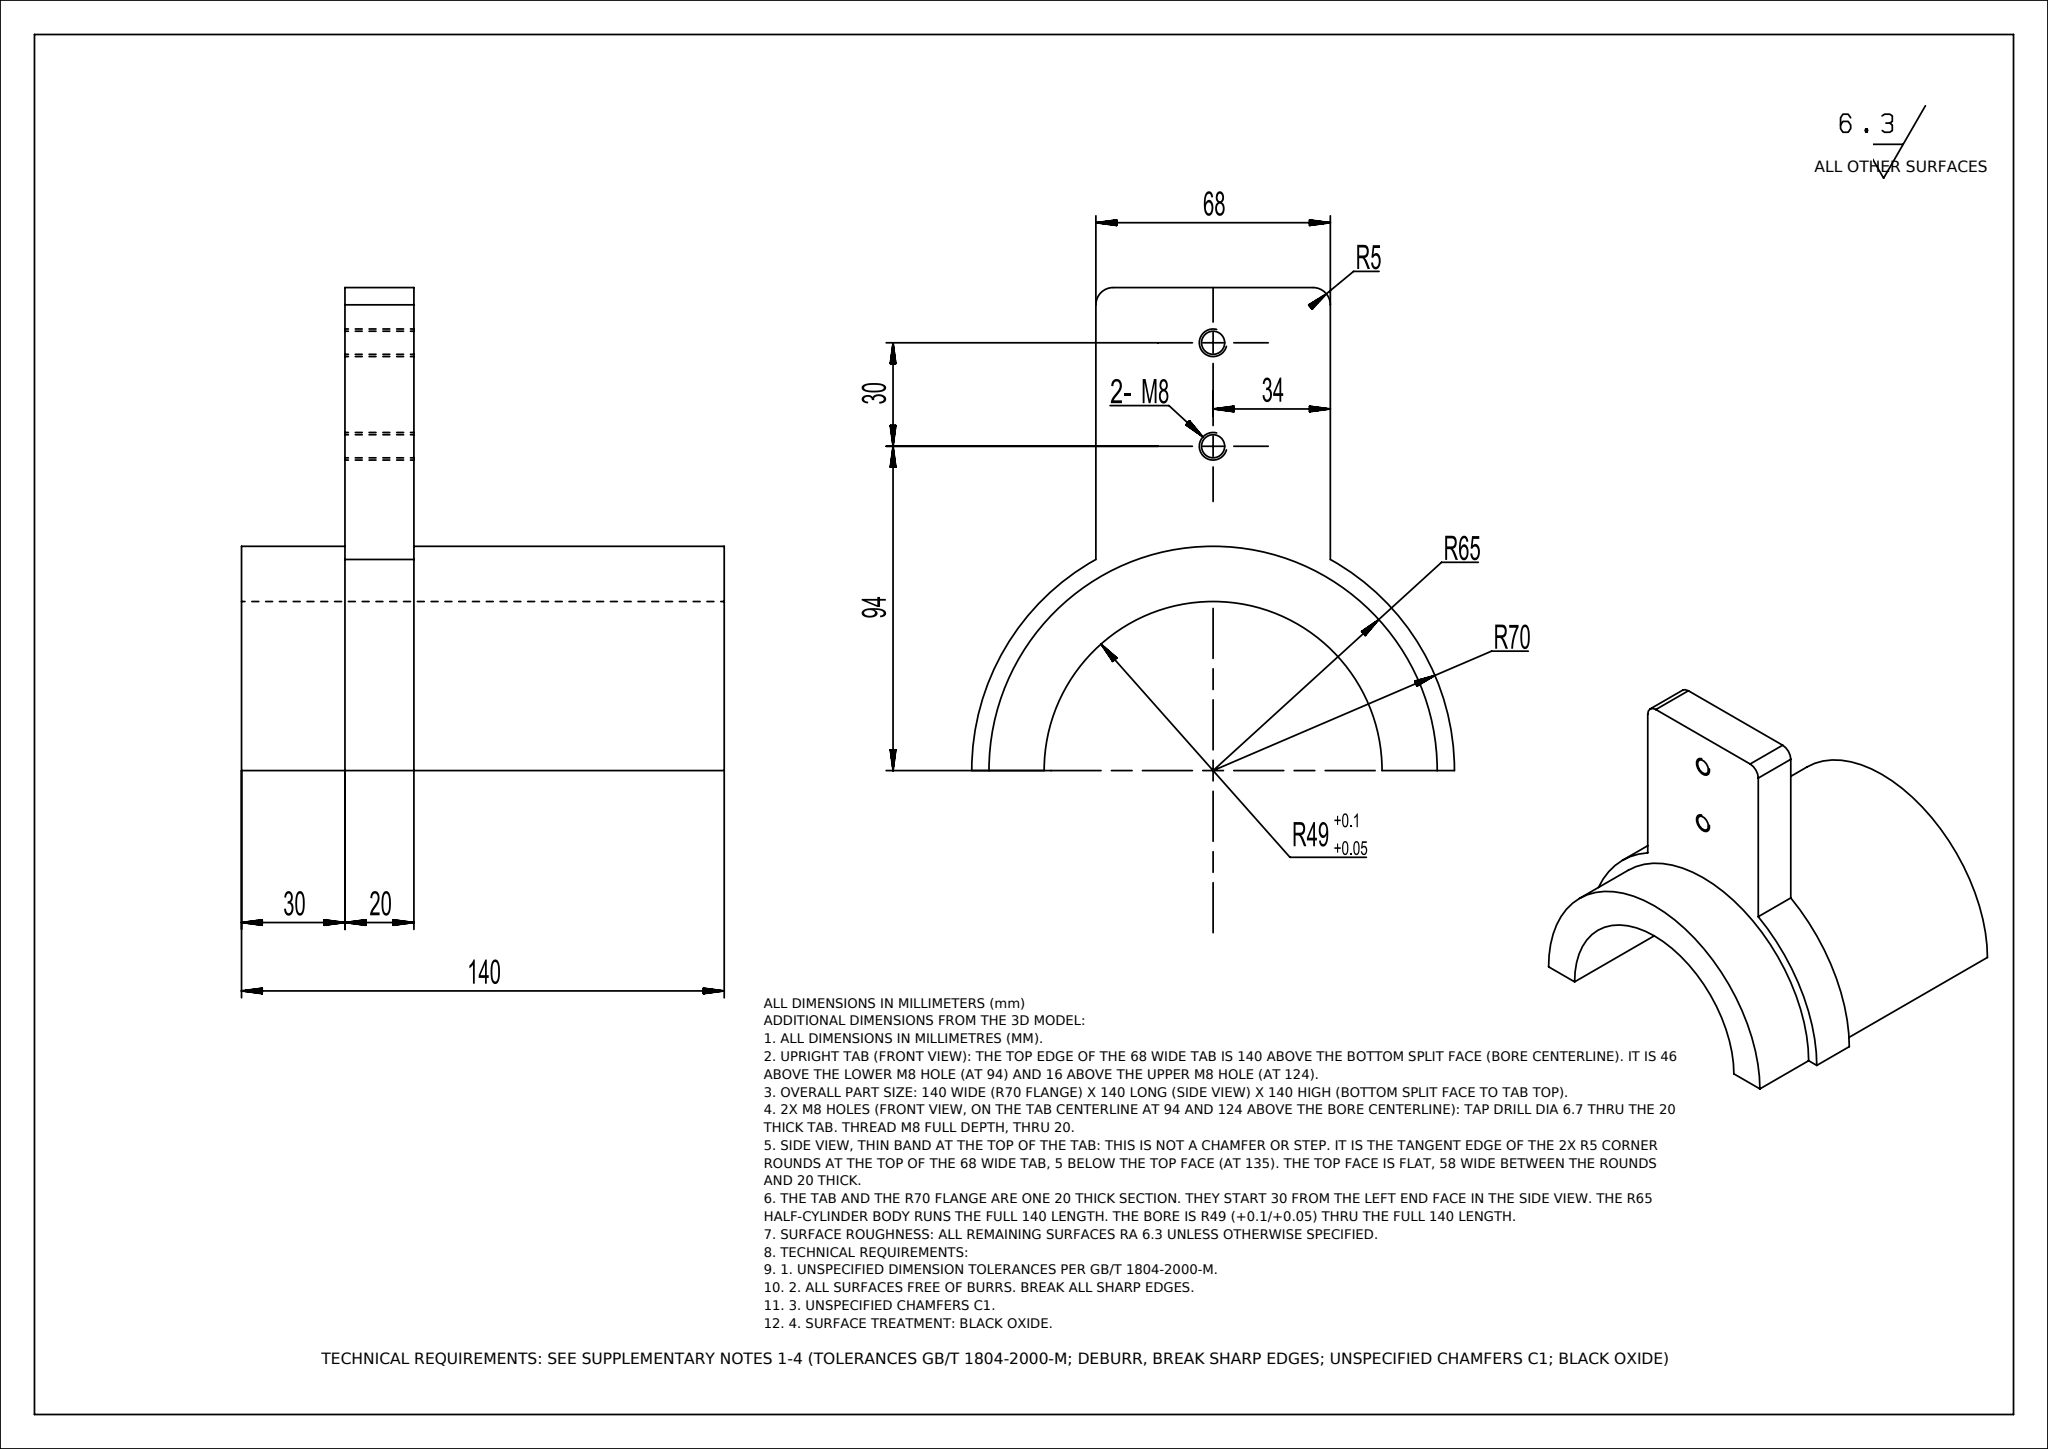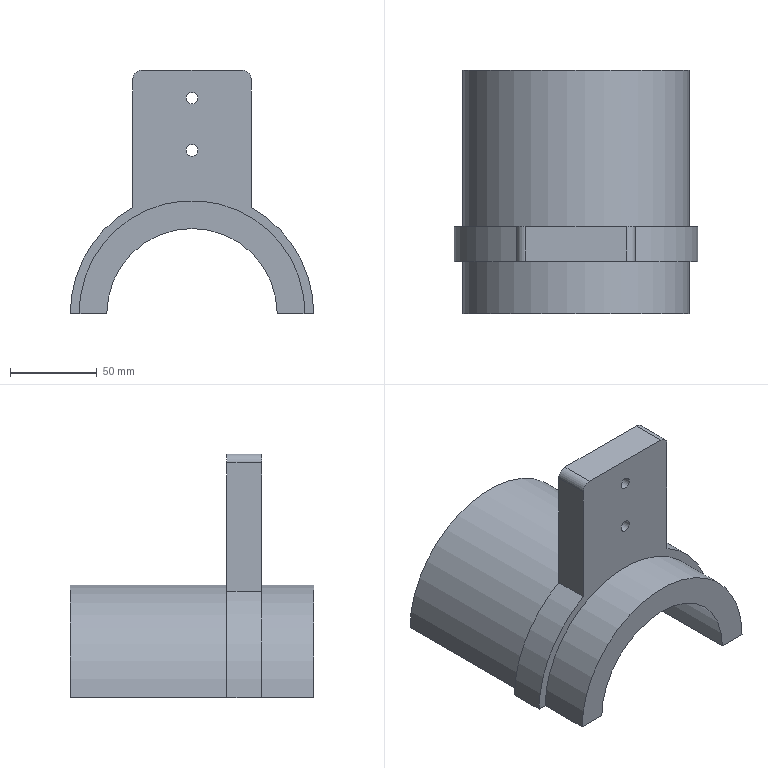Part | NX | mm | 1 solid | 18 faces | box 140 x 140 x 140 mm | volume 519788 mm3 | cylinder 9 | plane 9 | commonest cylinder face diameters 130 x2 140 x2 6.7 x2 10 x2 98 x1
STEP:
#1=CARTESIAN_POINT('',(0.,0.,0.));
#2=DIRECTION('',(0.,0.,1.));
#3=DIRECTION('',(1.,0.,0.));
#4=AXIS2_PLACEMENT_3D('',#1,#2,#3);
#5=(LENGTH_UNIT()NAMED_UNIT(*)SI_UNIT(.MILLI.,.METRE.));
#6=UNCERTAINTY_MEASURE_WITH_UNIT(LENGTH_MEASURE(0.00002),#5,'','');
#7=(NAMED_UNIT(*)PLANE_ANGLE_UNIT()SI_UNIT($,.RADIAN.));
#8=PLANE_ANGLE_MEASURE_WITH_UNIT(PLANE_ANGLE_MEASURE(0.01745),#7);
#9=DIMENSIONAL_EXPONENTS(0.,0.,0.,0.,0.,0.,0.);
#10=(CONVERSION_BASED_UNIT('',#8)NAMED_UNIT(#9)PLANE_ANGLE_UNIT());
#11=(NAMED_UNIT(*)SI_UNIT($,.STERADIAN.)SOLID_ANGLE_UNIT());
#12=(GEOMETRIC_REPRESENTATION_CONTEXT(3)GLOBAL_UNCERTAINTY_ASSIGNED_CONTEXT((#6))GLOBAL_UNIT_ASSIGNED_CONTEXT((#5,#10,#11))REPRESENTATION_CONTEXT('',''));
#13=SHAPE_REPRESENTATION('',(#4),#12);
#14=CARTESIAN_POINT('',(-65.,140.,0.));
#15=VERTEX_POINT('',#14);
#16=CARTESIAN_POINT('',(-65.,50.,0.));
#17=VERTEX_POINT('',#16);
#18=CARTESIAN_POINT('',(-65.,140.,0.));
#19=DIRECTION('',(0.,-1.,0.));
#20=VECTOR('',#19,1.);
#21=LINE('',#18,#20);
#22=EDGE_CURVE('',#15,#17,#21,.T.);
#23=ORIENTED_EDGE('',*,*,#22,.T.);
#24=CARTESIAN_POINT('',(65.,50.,0.));
#25=VERTEX_POINT('',#24);
#26=CARTESIAN_POINT('',(0.,50.,0.));
#27=DIRECTION('',(0.,1.,0.));
#28=DIRECTION('',(1.,0.,0.));
#29=AXIS2_PLACEMENT_3D('',#26,#27,#28);
#30=CIRCLE('',#29,65.);
#31=EDGE_CURVE('',#17,#25,#30,.T.);
#32=ORIENTED_EDGE('',*,*,#31,.T.);
#33=CARTESIAN_POINT('',(65.,140.,0.));
#34=VERTEX_POINT('',#33);
#35=CARTESIAN_POINT('',(65.,140.,0.));
#36=DIRECTION('',(0.,-1.,0.));
#37=VECTOR('',#36,1.);
#38=LINE('',#35,#37);
#39=EDGE_CURVE('',#34,#25,#38,.T.);
#40=ORIENTED_EDGE('',*,*,#39,.F.);
#41=CARTESIAN_POINT('',(0.,140.,0.));
#42=DIRECTION('',(0.,-1.,0.));
#43=DIRECTION('',(1.,0.,-0.));
#44=AXIS2_PLACEMENT_3D('',#41,#42,#43);
#45=CIRCLE('',#44,65.);
#46=EDGE_CURVE('',#34,#15,#45,.T.);
#47=ORIENTED_EDGE('',*,*,#46,.T.);
#48=EDGE_LOOP('',(#23,#32,#40,#47));
#49=FACE_OUTER_BOUND('',#48,.T.);
#50=CARTESIAN_POINT('',(0.,140.,0.));
#51=DIRECTION('',(0.,-1.,0.));
#52=DIRECTION('',(0.,0.,-1.));
#53=AXIS2_PLACEMENT_3D('',#50,#51,#52);
#54=CYLINDRICAL_SURFACE('',#53,65.);
#55=ADVANCED_FACE('',(#49),#54,.T.);
#56=CARTESIAN_POINT('',(-65.,0.,0.));
#57=VERTEX_POINT('',#56);
#58=CARTESIAN_POINT('',(-49.,0.,0.));
#59=VERTEX_POINT('',#58);
#60=CARTESIAN_POINT('',(-65.,0.,0.));
#61=DIRECTION('',(1.,0.,0.));
#62=VECTOR('',#61,1.);
#63=LINE('',#60,#62);
#64=EDGE_CURVE('',#57,#59,#63,.T.);
#65=ORIENTED_EDGE('',*,*,#64,.F.);
#66=CARTESIAN_POINT('',(-65.,30.,0.));
#67=VERTEX_POINT('',#66);
#68=CARTESIAN_POINT('',(-65.,140.,0.));
#69=DIRECTION('',(0.,-1.,0.));
#70=VECTOR('',#69,1.);
#71=LINE('',#68,#70);
#72=EDGE_CURVE('',#67,#57,#71,.T.);
#73=ORIENTED_EDGE('',*,*,#72,.F.);
#74=CARTESIAN_POINT('',(-70.,30.,0.));
#75=VERTEX_POINT('',#74);
#76=CARTESIAN_POINT('',(-70.,30.,0.));
#77=DIRECTION('',(1.,0.,0.));
#78=VECTOR('',#77,1.);
#79=LINE('',#76,#78);
#80=EDGE_CURVE('',#75,#67,#79,.T.);
#81=ORIENTED_EDGE('',*,*,#80,.F.);
#82=CARTESIAN_POINT('',(-70.,50.,0.));
#83=VERTEX_POINT('',#82);
#84=CARTESIAN_POINT('',(-70.,50.,0.));
#85=DIRECTION('',(0.,-1.,0.));
#86=VECTOR('',#85,1.);
#87=LINE('',#84,#86);
#88=EDGE_CURVE('',#83,#75,#87,.T.);
#89=ORIENTED_EDGE('',*,*,#88,.F.);
#90=CARTESIAN_POINT('',(-70.,50.,0.));
#91=DIRECTION('',(1.,0.,0.));
#92=VECTOR('',#91,1.);
#93=LINE('',#90,#92);
#94=EDGE_CURVE('',#83,#17,#93,.T.);
#95=ORIENTED_EDGE('',*,*,#94,.T.);
#96=ORIENTED_EDGE('',*,*,#22,.F.);
#97=CARTESIAN_POINT('',(-49.,140.,0.));
#98=VERTEX_POINT('',#97);
#99=CARTESIAN_POINT('',(-65.,140.,0.));
#100=DIRECTION('',(1.,0.,0.));
#101=VECTOR('',#100,1.);
#102=LINE('',#99,#101);
#103=EDGE_CURVE('',#15,#98,#102,.T.);
#104=ORIENTED_EDGE('',*,*,#103,.T.);
#105=CARTESIAN_POINT('',(-49.,140.,0.));
#106=DIRECTION('',(0.,-1.,0.));
#107=VECTOR('',#106,1.);
#108=LINE('',#105,#107);
#109=EDGE_CURVE('',#98,#59,#108,.T.);
#110=ORIENTED_EDGE('',*,*,#109,.T.);
#111=EDGE_LOOP('',(#65,#73,#81,#89,#95,#96,#104,#110));
#112=FACE_OUTER_BOUND('',#111,.T.);
#113=CARTESIAN_POINT('',(-65.,140.,0.));
#114=DIRECTION('',(0.,0.,-1.));
#115=DIRECTION('',(-1.,0.,-0.));
#116=AXIS2_PLACEMENT_3D('',#113,#114,#115);
#117=PLANE('',#116);
#118=ADVANCED_FACE('',(#112),#117,.T.);
#119=CARTESIAN_POINT('',(49.,0.,0.));
#120=VERTEX_POINT('',#119);
#121=CARTESIAN_POINT('',(0.,0.,0.));
#122=DIRECTION('',(0.,1.,0.));
#123=DIRECTION('',(1.,0.,0.));
#124=AXIS2_PLACEMENT_3D('',#121,#122,#123);
#125=CIRCLE('',#124,49.);
#126=EDGE_CURVE('',#59,#120,#125,.T.);
#127=ORIENTED_EDGE('',*,*,#126,.F.);
#128=ORIENTED_EDGE('',*,*,#109,.F.);
#129=CARTESIAN_POINT('',(49.,140.,0.));
#130=VERTEX_POINT('',#129);
#131=CARTESIAN_POINT('',(0.,140.,0.));
#132=DIRECTION('',(0.,1.,0.));
#133=DIRECTION('',(1.,0.,0.));
#134=AXIS2_PLACEMENT_3D('',#131,#132,#133);
#135=CIRCLE('',#134,49.);
#136=EDGE_CURVE('',#98,#130,#135,.T.);
#137=ORIENTED_EDGE('',*,*,#136,.T.);
#138=CARTESIAN_POINT('',(49.,140.,0.));
#139=DIRECTION('',(0.,-1.,0.));
#140=VECTOR('',#139,1.);
#141=LINE('',#138,#140);
#142=EDGE_CURVE('',#130,#120,#141,.T.);
#143=ORIENTED_EDGE('',*,*,#142,.T.);
#144=EDGE_LOOP('',(#127,#128,#137,#143));
#145=FACE_OUTER_BOUND('',#144,.T.);
#146=CARTESIAN_POINT('',(0.,140.,0.));
#147=DIRECTION('',(0.,-1.,0.));
#148=DIRECTION('',(0.,0.,-1.));
#149=AXIS2_PLACEMENT_3D('',#146,#147,#148);
#150=CYLINDRICAL_SURFACE('',#149,49.);
#151=ADVANCED_FACE('',(#145),#150,.F.);
#152=CARTESIAN_POINT('',(65.,0.,0.));
#153=VERTEX_POINT('',#152);
#154=CARTESIAN_POINT('',(49.,0.,0.));
#155=DIRECTION('',(1.,0.,0.));
#156=VECTOR('',#155,1.);
#157=LINE('',#154,#156);
#158=EDGE_CURVE('',#120,#153,#157,.T.);
#159=ORIENTED_EDGE('',*,*,#158,.F.);
#160=ORIENTED_EDGE('',*,*,#142,.F.);
#161=CARTESIAN_POINT('',(49.,140.,0.));
#162=DIRECTION('',(1.,0.,0.));
#163=VECTOR('',#162,1.);
#164=LINE('',#161,#163);
#165=EDGE_CURVE('',#130,#34,#164,.T.);
#166=ORIENTED_EDGE('',*,*,#165,.T.);
#167=ORIENTED_EDGE('',*,*,#39,.T.);
#168=CARTESIAN_POINT('',(70.,50.,-0.));
#169=VERTEX_POINT('',#168);
#170=CARTESIAN_POINT('',(65.,50.,0.));
#171=DIRECTION('',(1.,0.,-0.));
#172=VECTOR('',#171,1.);
#173=LINE('',#170,#172);
#174=EDGE_CURVE('',#25,#169,#173,.T.);
#175=ORIENTED_EDGE('',*,*,#174,.T.);
#176=CARTESIAN_POINT('',(70.,30.,-0.));
#177=VERTEX_POINT('',#176);
#178=CARTESIAN_POINT('',(70.,50.,-0.));
#179=DIRECTION('',(0.,-1.,0.));
#180=VECTOR('',#179,1.);
#181=LINE('',#178,#180);
#182=EDGE_CURVE('',#169,#177,#181,.T.);
#183=ORIENTED_EDGE('',*,*,#182,.T.);
#184=CARTESIAN_POINT('',(65.,30.,0.));
#185=VERTEX_POINT('',#184);
#186=CARTESIAN_POINT('',(65.,30.,0.));
#187=DIRECTION('',(1.,0.,-0.));
#188=VECTOR('',#187,1.);
#189=LINE('',#186,#188);
#190=EDGE_CURVE('',#185,#177,#189,.T.);
#191=ORIENTED_EDGE('',*,*,#190,.F.);
#192=CARTESIAN_POINT('',(65.,140.,0.));
#193=DIRECTION('',(0.,-1.,0.));
#194=VECTOR('',#193,1.);
#195=LINE('',#192,#194);
#196=EDGE_CURVE('',#185,#153,#195,.T.);
#197=ORIENTED_EDGE('',*,*,#196,.T.);
#198=EDGE_LOOP('',(#159,#160,#166,#167,#175,#183,#191,#197));
#199=FACE_OUTER_BOUND('',#198,.T.);
#200=CARTESIAN_POINT('',(49.,140.,0.));
#201=DIRECTION('',(0.,0.,-1.));
#202=DIRECTION('',(-1.,0.,-0.));
#203=AXIS2_PLACEMENT_3D('',#200,#201,#202);
#204=PLANE('',#203);
#205=ADVANCED_FACE('',(#199),#204,.T.);
#206=CARTESIAN_POINT('',(0.,30.,0.));
#207=DIRECTION('',(0.,1.,0.));
#208=DIRECTION('',(1.,0.,0.));
#209=AXIS2_PLACEMENT_3D('',#206,#207,#208);
#210=CIRCLE('',#209,65.);
#211=EDGE_CURVE('',#67,#185,#210,.T.);
#212=ORIENTED_EDGE('',*,*,#211,.F.);
#213=ORIENTED_EDGE('',*,*,#72,.T.);
#214=CARTESIAN_POINT('',(0.,0.,0.));
#215=DIRECTION('',(0.,-1.,0.));
#216=DIRECTION('',(1.,0.,-0.));
#217=AXIS2_PLACEMENT_3D('',#214,#215,#216);
#218=CIRCLE('',#217,65.);
#219=EDGE_CURVE('',#153,#57,#218,.T.);
#220=ORIENTED_EDGE('',*,*,#219,.F.);
#221=ORIENTED_EDGE('',*,*,#196,.F.);
#222=EDGE_LOOP('',(#212,#213,#220,#221));
#223=FACE_OUTER_BOUND('',#222,.T.);
#224=CARTESIAN_POINT('',(0.,140.,0.));
#225=DIRECTION('',(0.,-1.,0.));
#226=DIRECTION('',(0.,0.,-1.));
#227=AXIS2_PLACEMENT_3D('',#224,#225,#226);
#228=CYLINDRICAL_SURFACE('',#227,65.);
#229=ADVANCED_FACE('',(#223),#228,.T.);
#230=ORIENTED_EDGE('',*,*,#103,.F.);
#231=ORIENTED_EDGE('',*,*,#46,.F.);
#232=ORIENTED_EDGE('',*,*,#165,.F.);
#233=ORIENTED_EDGE('',*,*,#136,.F.);
#234=EDGE_LOOP('',(#230,#231,#232,#233));
#235=FACE_OUTER_BOUND('',#234,.T.);
#236=CARTESIAN_POINT('',(0.,140.,0.));
#237=DIRECTION('',(0.,1.,0.));
#238=DIRECTION('',(0.,0.,1.));
#239=AXIS2_PLACEMENT_3D('',#236,#237,#238);
#240=PLANE('',#239);
#241=ADVANCED_FACE('',(#235),#240,.T.);
#242=ORIENTED_EDGE('',*,*,#64,.T.);
#243=ORIENTED_EDGE('',*,*,#126,.T.);
#244=ORIENTED_EDGE('',*,*,#158,.T.);
#245=ORIENTED_EDGE('',*,*,#219,.T.);
#246=EDGE_LOOP('',(#242,#243,#244,#245));
#247=FACE_OUTER_BOUND('',#246,.T.);
#248=CARTESIAN_POINT('',(0.,0.,0.));
#249=DIRECTION('',(0.,1.,0.));
#250=DIRECTION('',(0.,0.,1.));
#251=AXIS2_PLACEMENT_3D('',#248,#249,#250);
#252=PLANE('',#251);
#253=ADVANCED_FACE('',(#247),#252,.F.);
#254=CARTESIAN_POINT('',(34.,30.,61.188));
#255=VERTEX_POINT('',#254);
#256=CARTESIAN_POINT('',(0.,30.,0.));
#257=DIRECTION('',(0.,-1.,0.));
#258=DIRECTION('',(1.,0.,-0.));
#259=AXIS2_PLACEMENT_3D('',#256,#257,#258);
#260=CIRCLE('',#259,70.);
#261=EDGE_CURVE('',#177,#255,#260,.T.);
#262=ORIENTED_EDGE('',*,*,#261,.F.);
#263=ORIENTED_EDGE('',*,*,#182,.F.);
#264=CARTESIAN_POINT('',(34.,50.,61.188));
#265=VERTEX_POINT('',#264);
#266=CARTESIAN_POINT('',(0.,50.,0.));
#267=DIRECTION('',(0.,-1.,0.));
#268=DIRECTION('',(1.,0.,-0.));
#269=AXIS2_PLACEMENT_3D('',#266,#267,#268);
#270=CIRCLE('',#269,70.);
#271=EDGE_CURVE('',#169,#265,#270,.T.);
#272=ORIENTED_EDGE('',*,*,#271,.T.);
#273=CARTESIAN_POINT('',(34.,50.,61.188));
#274=DIRECTION('',(0.,-1.,0.));
#275=VECTOR('',#274,1.);
#276=LINE('',#273,#275);
#277=EDGE_CURVE('',#265,#255,#276,.T.);
#278=ORIENTED_EDGE('',*,*,#277,.T.);
#279=EDGE_LOOP('',(#262,#263,#272,#278));
#280=FACE_OUTER_BOUND('',#279,.T.);
#281=CARTESIAN_POINT('',(0.,50.,0.));
#282=DIRECTION('',(0.,-1.,0.));
#283=DIRECTION('',(0.,0.,-1.));
#284=AXIS2_PLACEMENT_3D('',#281,#282,#283);
#285=CYLINDRICAL_SURFACE('',#284,70.);
#286=ADVANCED_FACE('',(#280),#285,.T.);
#287=CARTESIAN_POINT('',(34.,50.,135.));
#288=VERTEX_POINT('',#287);
#289=CARTESIAN_POINT('',(34.,50.,61.188));
#290=DIRECTION('',(-0.,0.,1.));
#291=VECTOR('',#290,1.);
#292=LINE('',#289,#291);
#293=EDGE_CURVE('',#265,#288,#292,.T.);
#294=ORIENTED_EDGE('',*,*,#293,.T.);
#295=CARTESIAN_POINT('',(34.,30.,135.));
#296=VERTEX_POINT('',#295);
#297=CARTESIAN_POINT('',(34.,50.,135.));
#298=DIRECTION('',(0.,-1.,0.));
#299=VECTOR('',#298,1.);
#300=LINE('',#297,#299);
#301=EDGE_CURVE('',#288,#296,#300,.T.);
#302=ORIENTED_EDGE('',*,*,#301,.T.);
#303=CARTESIAN_POINT('',(34.,30.,61.188));
#304=DIRECTION('',(-0.,0.,1.));
#305=VECTOR('',#304,1.);
#306=LINE('',#303,#305);
#307=EDGE_CURVE('',#255,#296,#306,.T.);
#308=ORIENTED_EDGE('',*,*,#307,.F.);
#309=ORIENTED_EDGE('',*,*,#277,.F.);
#310=EDGE_LOOP('',(#294,#302,#308,#309));
#311=FACE_OUTER_BOUND('',#310,.T.);
#312=CARTESIAN_POINT('',(34.,50.,61.188));
#313=DIRECTION('',(1.,0.,0.));
#314=DIRECTION('',(0.,0.,-1.));
#315=AXIS2_PLACEMENT_3D('',#312,#313,#314);
#316=PLANE('',#315);
#317=ADVANCED_FACE('',(#311),#316,.T.);
#318=CARTESIAN_POINT('',(29.,50.,140.));
#319=VERTEX_POINT('',#318);
#320=CARTESIAN_POINT('',(-29.,50.,140.));
#321=VERTEX_POINT('',#320);
#322=CARTESIAN_POINT('',(34.,50.,140.));
#323=DIRECTION('',(-1.,0.,0.));
#324=VECTOR('',#323,1.);
#325=LINE('',#322,#324);
#326=EDGE_CURVE('',#319,#321,#325,.T.);
#327=ORIENTED_EDGE('',*,*,#326,.T.);
#328=CARTESIAN_POINT('',(-29.,30.,140.));
#329=VERTEX_POINT('',#328);
#330=CARTESIAN_POINT('',(-29.,50.,140.));
#331=DIRECTION('',(0.,-1.,0.));
#332=VECTOR('',#331,1.);
#333=LINE('',#330,#332);
#334=EDGE_CURVE('',#321,#329,#333,.T.);
#335=ORIENTED_EDGE('',*,*,#334,.T.);
#336=CARTESIAN_POINT('',(29.,30.,140.));
#337=VERTEX_POINT('',#336);
#338=CARTESIAN_POINT('',(34.,30.,140.));
#339=DIRECTION('',(-1.,0.,0.));
#340=VECTOR('',#339,1.);
#341=LINE('',#338,#340);
#342=EDGE_CURVE('',#337,#329,#341,.T.);
#343=ORIENTED_EDGE('',*,*,#342,.F.);
#344=CARTESIAN_POINT('',(29.,50.,140.));
#345=DIRECTION('',(0.,1.,0.));
#346=VECTOR('',#345,1.);
#347=LINE('',#344,#346);
#348=EDGE_CURVE('',#337,#319,#347,.T.);
#349=ORIENTED_EDGE('',*,*,#348,.T.);
#350=EDGE_LOOP('',(#327,#335,#343,#349));
#351=FACE_OUTER_BOUND('',#350,.T.);
#352=CARTESIAN_POINT('',(34.,50.,140.));
#353=DIRECTION('',(0.,0.,1.));
#354=DIRECTION('',(1.,0.,0.));
#355=AXIS2_PLACEMENT_3D('',#352,#353,#354);
#356=PLANE('',#355);
#357=ADVANCED_FACE('',(#351),#356,.T.);
#358=CARTESIAN_POINT('',(-34.,30.,135.));
#359=VERTEX_POINT('',#358);
#360=CARTESIAN_POINT('',(-34.,30.,61.188));
#361=VERTEX_POINT('',#360);
#362=CARTESIAN_POINT('',(-34.,30.,140.));
#363=DIRECTION('',(-0.,0.,-1.));
#364=VECTOR('',#363,1.);
#365=LINE('',#362,#364);
#366=EDGE_CURVE('',#359,#361,#365,.T.);
#367=ORIENTED_EDGE('',*,*,#366,.F.);
#368=CARTESIAN_POINT('',(-34.,50.,135.));
#369=VERTEX_POINT('',#368);
#370=CARTESIAN_POINT('',(-34.,50.,135.));
#371=DIRECTION('',(0.,1.,0.));
#372=VECTOR('',#371,1.);
#373=LINE('',#370,#372);
#374=EDGE_CURVE('',#359,#369,#373,.T.);
#375=ORIENTED_EDGE('',*,*,#374,.T.);
#376=CARTESIAN_POINT('',(-34.,50.,61.188));
#377=VERTEX_POINT('',#376);
#378=CARTESIAN_POINT('',(-34.,50.,140.));
#379=DIRECTION('',(-0.,0.,-1.));
#380=VECTOR('',#379,1.);
#381=LINE('',#378,#380);
#382=EDGE_CURVE('',#369,#377,#381,.T.);
#383=ORIENTED_EDGE('',*,*,#382,.T.);
#384=CARTESIAN_POINT('',(-34.,50.,61.188));
#385=DIRECTION('',(0.,-1.,0.));
#386=VECTOR('',#385,1.);
#387=LINE('',#384,#386);
#388=EDGE_CURVE('',#377,#361,#387,.T.);
#389=ORIENTED_EDGE('',*,*,#388,.T.);
#390=EDGE_LOOP('',(#367,#375,#383,#389));
#391=FACE_OUTER_BOUND('',#390,.T.);
#392=CARTESIAN_POINT('',(-34.,50.,140.));
#393=DIRECTION('',(-1.,0.,0.));
#394=DIRECTION('',(0.,0.,1.));
#395=AXIS2_PLACEMENT_3D('',#392,#393,#394);
#396=PLANE('',#395);
#397=ADVANCED_FACE('',(#391),#396,.T.);
#398=CARTESIAN_POINT('',(3.35,50.,94.));
#399=VERTEX_POINT('',#398);
#400=CARTESIAN_POINT('',(0.,50.,94.));
#401=DIRECTION('',(0.,-1.,0.));
#402=DIRECTION('',(1.,0.,0.));
#403=AXIS2_PLACEMENT_3D('',#400,#401,#402);
#404=CIRCLE('',#403,3.35);
#405=EDGE_CURVE('',#399,#399,#404,.T.);
#406=ORIENTED_EDGE('',*,*,#405,.F.);
#407=EDGE_LOOP('',(#406));
#408=FACE_BOUND('',#407,.T.);
#409=CARTESIAN_POINT('',(3.35,30.,94.));
#410=VERTEX_POINT('',#409);
#411=CARTESIAN_POINT('',(0.,30.,94.));
#412=DIRECTION('',(0.,-1.,0.));
#413=DIRECTION('',(1.,0.,0.));
#414=AXIS2_PLACEMENT_3D('',#411,#412,#413);
#415=CIRCLE('',#414,3.35);
#416=EDGE_CURVE('',#410,#410,#415,.T.);
#417=ORIENTED_EDGE('',*,*,#416,.T.);
#418=EDGE_LOOP('',(#417));
#419=FACE_BOUND('',#418,.T.);
#420=CARTESIAN_POINT('',(0.,50.,94.));
#421=DIRECTION('',(0.,-1.,0.));
#422=DIRECTION('',(0.,0.,-1.));
#423=AXIS2_PLACEMENT_3D('',#420,#421,#422);
#424=CYLINDRICAL_SURFACE('',#423,3.35);
#425=ADVANCED_FACE('',(#408,#419),#424,.F.);
#426=CARTESIAN_POINT('',(0.,30.,0.));
#427=DIRECTION('',(0.,-1.,0.));
#428=DIRECTION('',(1.,0.,-0.));
#429=AXIS2_PLACEMENT_3D('',#426,#427,#428);
#430=CIRCLE('',#429,70.);
#431=EDGE_CURVE('',#361,#75,#430,.T.);
#432=ORIENTED_EDGE('',*,*,#431,.F.);
#433=ORIENTED_EDGE('',*,*,#388,.F.);
#434=CARTESIAN_POINT('',(0.,50.,0.));
#435=DIRECTION('',(0.,-1.,0.));
#436=DIRECTION('',(1.,0.,-0.));
#437=AXIS2_PLACEMENT_3D('',#434,#435,#436);
#438=CIRCLE('',#437,70.);
#439=EDGE_CURVE('',#377,#83,#438,.T.);
#440=ORIENTED_EDGE('',*,*,#439,.T.);
#441=ORIENTED_EDGE('',*,*,#88,.T.);
#442=EDGE_LOOP('',(#432,#433,#440,#441));
#443=FACE_OUTER_BOUND('',#442,.T.);
#444=CARTESIAN_POINT('',(0.,50.,0.));
#445=DIRECTION('',(0.,-1.,0.));
#446=DIRECTION('',(0.,0.,-1.));
#447=AXIS2_PLACEMENT_3D('',#444,#445,#446);
#448=CYLINDRICAL_SURFACE('',#447,70.);
#449=ADVANCED_FACE('',(#443),#448,.T.);
#450=CARTESIAN_POINT('',(3.35,50.,124.));
#451=VERTEX_POINT('',#450);
#452=CARTESIAN_POINT('',(0.,50.,124.));
#453=DIRECTION('',(0.,-1.,0.));
#454=DIRECTION('',(1.,0.,0.));
#455=AXIS2_PLACEMENT_3D('',#452,#453,#454);
#456=CIRCLE('',#455,3.35);
#457=EDGE_CURVE('',#451,#451,#456,.T.);
#458=ORIENTED_EDGE('',*,*,#457,.F.);
#459=EDGE_LOOP('',(#458));
#460=FACE_BOUND('',#459,.T.);
#461=CARTESIAN_POINT('',(3.35,30.,124.));
#462=VERTEX_POINT('',#461);
#463=CARTESIAN_POINT('',(0.,30.,124.));
#464=DIRECTION('',(0.,-1.,0.));
#465=DIRECTION('',(1.,0.,0.));
#466=AXIS2_PLACEMENT_3D('',#463,#464,#465);
#467=CIRCLE('',#466,3.35);
#468=EDGE_CURVE('',#462,#462,#467,.T.);
#469=ORIENTED_EDGE('',*,*,#468,.T.);
#470=EDGE_LOOP('',(#469));
#471=FACE_BOUND('',#470,.T.);
#472=CARTESIAN_POINT('',(0.,50.,124.));
#473=DIRECTION('',(0.,-1.,0.));
#474=DIRECTION('',(0.,0.,-1.));
#475=AXIS2_PLACEMENT_3D('',#472,#473,#474);
#476=CYLINDRICAL_SURFACE('',#475,3.35);
#477=ADVANCED_FACE('',(#460,#471),#476,.F.);
#478=ORIENTED_EDGE('',*,*,#382,.F.);
#479=CARTESIAN_POINT('',(-29.,50.,135.));
#480=DIRECTION('',(0.,1.,0.));
#481=DIRECTION('',(0.,0.,1.));
#482=AXIS2_PLACEMENT_3D('',#479,#480,#481);
#483=CIRCLE('',#482,5.);
#484=EDGE_CURVE('',#369,#321,#483,.T.);
#485=ORIENTED_EDGE('',*,*,#484,.T.);
#486=ORIENTED_EDGE('',*,*,#326,.F.);
#487=CARTESIAN_POINT('',(29.,50.,135.));
#488=DIRECTION('',(0.,1.,0.));
#489=DIRECTION('',(0.,0.,1.));
#490=AXIS2_PLACEMENT_3D('',#487,#488,#489);
#491=CIRCLE('',#490,5.);
#492=EDGE_CURVE('',#319,#288,#491,.T.);
#493=ORIENTED_EDGE('',*,*,#492,.T.);
#494=ORIENTED_EDGE('',*,*,#293,.F.);
#495=ORIENTED_EDGE('',*,*,#271,.F.);
#496=ORIENTED_EDGE('',*,*,#174,.F.);
#497=ORIENTED_EDGE('',*,*,#31,.F.);
#498=ORIENTED_EDGE('',*,*,#94,.F.);
#499=ORIENTED_EDGE('',*,*,#439,.F.);
#500=EDGE_LOOP('',(#478,#485,#486,#493,#494,#495,#496,#497,#498,#499));
#501=FACE_BOUND('',#500,.T.);
#502=ORIENTED_EDGE('',*,*,#405,.T.);
#503=EDGE_LOOP('',(#502));
#504=FACE_BOUND('',#503,.T.);
#505=ORIENTED_EDGE('',*,*,#457,.T.);
#506=EDGE_LOOP('',(#505));
#507=FACE_BOUND('',#506,.T.);
#508=CARTESIAN_POINT('',(0.,50.,0.));
#509=DIRECTION('',(0.,1.,0.));
#510=DIRECTION('',(0.,0.,1.));
#511=AXIS2_PLACEMENT_3D('',#508,#509,#510);
#512=PLANE('',#511);
#513=ADVANCED_FACE('',(#501,#504,#507),#512,.T.);
#514=ORIENTED_EDGE('',*,*,#342,.T.);
#515=CARTESIAN_POINT('',(-29.,30.,135.));
#516=DIRECTION('',(0.,-1.,0.));
#517=DIRECTION('',(0.,0.,1.));
#518=AXIS2_PLACEMENT_3D('',#515,#516,#517);
#519=CIRCLE('',#518,5.);
#520=EDGE_CURVE('',#329,#359,#519,.T.);
#521=ORIENTED_EDGE('',*,*,#520,.T.);
#522=ORIENTED_EDGE('',*,*,#366,.T.);
#523=ORIENTED_EDGE('',*,*,#431,.T.);
#524=ORIENTED_EDGE('',*,*,#80,.T.);
#525=ORIENTED_EDGE('',*,*,#211,.T.);
#526=ORIENTED_EDGE('',*,*,#190,.T.);
#527=ORIENTED_EDGE('',*,*,#261,.T.);
#528=ORIENTED_EDGE('',*,*,#307,.T.);
#529=CARTESIAN_POINT('',(29.,30.,135.));
#530=DIRECTION('',(0.,-1.,0.));
#531=DIRECTION('',(0.,0.,1.));
#532=AXIS2_PLACEMENT_3D('',#529,#530,#531);
#533=CIRCLE('',#532,5.);
#534=EDGE_CURVE('',#296,#337,#533,.T.);
#535=ORIENTED_EDGE('',*,*,#534,.T.);
#536=EDGE_LOOP('',(#514,#521,#522,#523,#524,#525,#526,#527,#528,#535));
#537=FACE_BOUND('',#536,.T.);
#538=ORIENTED_EDGE('',*,*,#416,.F.);
#539=EDGE_LOOP('',(#538));
#540=FACE_BOUND('',#539,.T.);
#541=ORIENTED_EDGE('',*,*,#468,.F.);
#542=EDGE_LOOP('',(#541));
#543=FACE_BOUND('',#542,.T.);
#544=CARTESIAN_POINT('',(0.,30.,0.));
#545=DIRECTION('',(0.,1.,0.));
#546=DIRECTION('',(0.,0.,1.));
#547=AXIS2_PLACEMENT_3D('',#544,#545,#546);
#548=PLANE('',#547);
#549=ADVANCED_FACE('',(#537,#540,#543),#548,.F.);
#550=ORIENTED_EDGE('',*,*,#484,.F.);
#551=ORIENTED_EDGE('',*,*,#374,.F.);
#552=ORIENTED_EDGE('',*,*,#520,.F.);
#553=ORIENTED_EDGE('',*,*,#334,.F.);
#554=EDGE_LOOP('',(#550,#551,#552,#553));
#555=FACE_OUTER_BOUND('',#554,.T.);
#556=CARTESIAN_POINT('',(-29.,50.,135.));
#557=DIRECTION('',(0.,-1.,0.));
#558=DIRECTION('',(0.,0.,-1.));
#559=AXIS2_PLACEMENT_3D('',#556,#557,#558);
#560=CYLINDRICAL_SURFACE('',#559,5.);
#561=ADVANCED_FACE('',(#555),#560,.T.);
#562=ORIENTED_EDGE('',*,*,#492,.F.);
#563=ORIENTED_EDGE('',*,*,#348,.F.);
#564=ORIENTED_EDGE('',*,*,#534,.F.);
#565=ORIENTED_EDGE('',*,*,#301,.F.);
#566=EDGE_LOOP('',(#562,#563,#564,#565));
#567=FACE_OUTER_BOUND('',#566,.T.);
#568=CARTESIAN_POINT('',(29.,50.,135.));
#569=DIRECTION('',(0.,-1.,0.));
#570=DIRECTION('',(0.,0.,-1.));
#571=AXIS2_PLACEMENT_3D('',#568,#569,#570);
#572=CYLINDRICAL_SURFACE('',#571,5.);
#573=ADVANCED_FACE('',(#567),#572,.T.);
#574=CLOSED_SHELL('',(#55,#118,#151,#205,#229,#241,#253,#286,#317,#357,#397,#425,#449,#477,#513,#549,#561,#573));
#575=MANIFOLD_SOLID_BREP('',#574);
#576=ADVANCED_BREP_SHAPE_REPRESENTATION('',(#575),#12);
#577=SHAPE_REPRESENTATION_RELATIONSHIP('','',#13,#576);
#578=PRESENTATION_LAYER_ASSIGNMENT('','',(#575));
#579=COLOUR_RGB('',1.,0.6,0.);
#580=FILL_AREA_STYLE_COLOUR('',#579);
#581=FILL_AREA_STYLE('',(#580));
#582=SURFACE_STYLE_FILL_AREA(#581);
#583=SURFACE_SIDE_STYLE('',(#582));
#584=SURFACE_STYLE_USAGE(.BOTH.,#583);
#585=PRESENTATION_STYLE_ASSIGNMENT((#584));
#586=STYLED_ITEM('',(#585),#575);
#587=MECHANICAL_DESIGN_GEOMETRIC_PRESENTATION_REPRESENTATION('',(#586),#12);